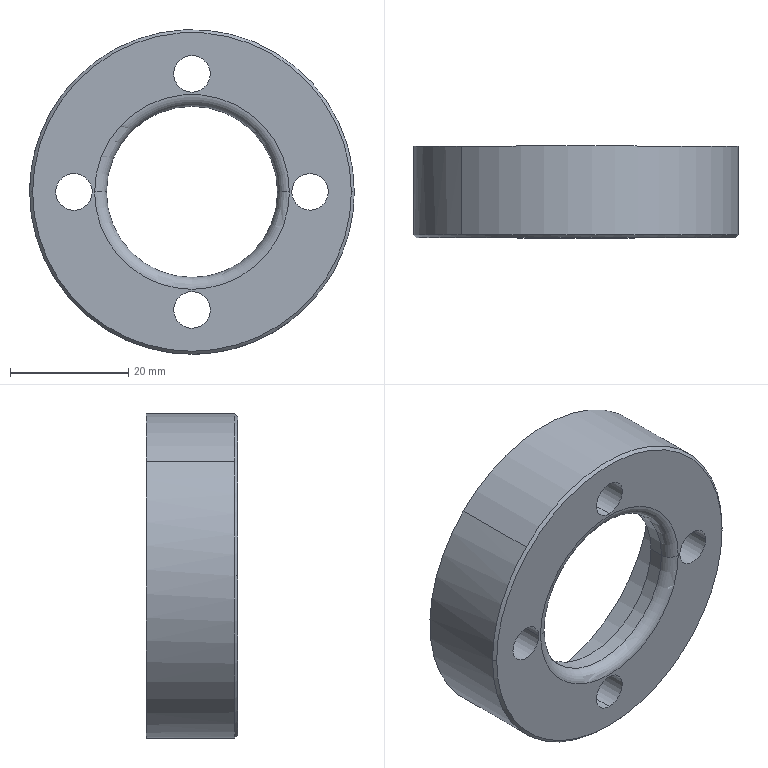CAM job | Mastercam | mm | 1 operations | part box 55 x 15.5 x 55
1. Drill/Counterbore | 7 - 4 倒角刀